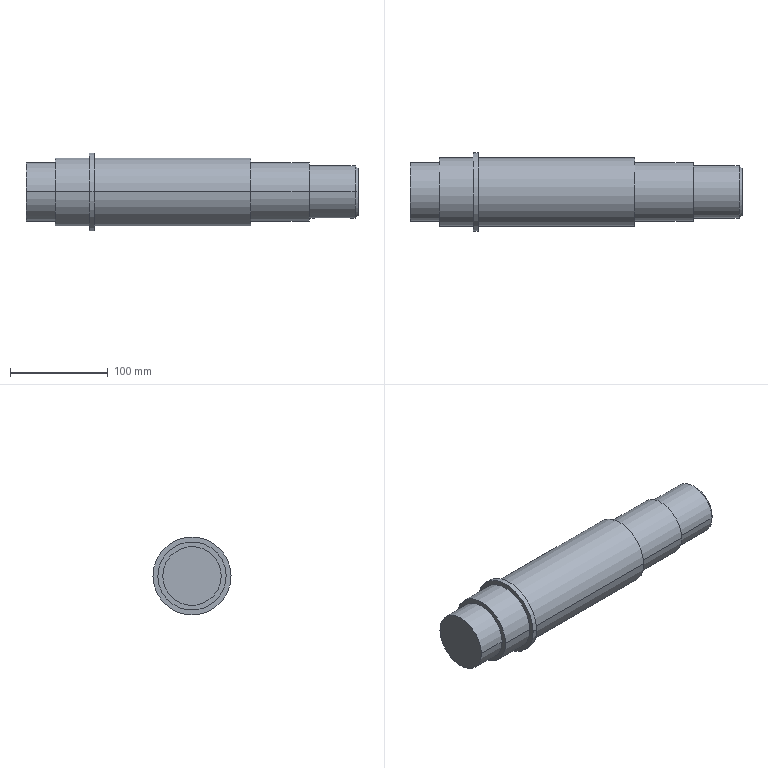Component | SolidWorks | TurbineShaft-1 | 1 solid | 28 faces | box 340 x 80 x 80 mm | volume 1142290 mm3 | cylinder 16 | plane 10 | cone 2 | commonest cylinder face diameters 60 x4 70 x4 10 x4 54 x2 80 x2
STEP:
#1=COLOUR_RGB('',0.7922,0.8196,0.9333);
#2=FILL_AREA_STYLE_COLOUR('',#1);
#3=FILL_AREA_STYLE('',(#2));
#4=SURFACE_STYLE_FILL_AREA(#3);
#5=SURFACE_SIDE_STYLE('',(#4));
#6=SURFACE_STYLE_USAGE(.BOTH.,#5);
#7=PRESENTATION_STYLE_ASSIGNMENT((#6));
#8=CARTESIAN_POINT('',(6.676,-1.282,-6.483));
#9=VERTEX_POINT('',#8);
#10=CARTESIAN_POINT('',(6.676,0.6077,-6.509));
#11=VERTEX_POINT('',#10);
#12=CARTESIAN_POINT('',(6.676,-0.3371,-6.496));
#13=DIRECTION('',(1.,0.,0.));
#14=DIRECTION('',(0.,0.9999,-0.01398));
#15=AXIS2_PLACEMENT_3D('',#12,#13,#14);
#16=CIRCLE('',#15,0.9449);
#17=EDGE_CURVE('',#9,#11,#16,.T.);
#18=ORIENTED_EDGE('',*,*,#17,.F.);
#19=CARTESIAN_POINT('',(6.558,-1.4,-6.481));
#20=VERTEX_POINT('',#19);
#21=CARTESIAN_POINT('',(6.558,-1.4,-6.481));
#22=DIRECTION('',(-0.7071,-0.707,0.009885));
#23=VECTOR('',#22,39.37);
#24=LINE('',#21,#23);
#25=EDGE_CURVE('',#9,#20,#24,.T.);
#26=ORIENTED_EDGE('',*,*,#25,.T.);
#27=CARTESIAN_POINT('',(6.558,0.7258,-6.511));
#28=VERTEX_POINT('',#27);
#29=CARTESIAN_POINT('',(6.558,-0.3371,-6.496));
#30=DIRECTION('',(-1.,-0.,-0.));
#31=DIRECTION('',(0.,0.9999,-0.01398));
#32=AXIS2_PLACEMENT_3D('',#29,#30,#31);
#33=CIRCLE('',#32,1.063);
#34=EDGE_CURVE('',#28,#20,#33,.T.);
#35=ORIENTED_EDGE('',*,*,#34,.F.);
#36=CARTESIAN_POINT('',(6.558,0.7258,-6.511));
#37=DIRECTION('',(-0.7071,0.707,-0.009885));
#38=VECTOR('',#37,39.37);
#39=LINE('',#36,#38);
#40=EDGE_CURVE('',#11,#28,#39,.T.);
#41=ORIENTED_EDGE('',*,*,#40,.F.);
#42=EDGE_LOOP('',(#18,#26,#35,#41));
#43=FACE_OUTER_BOUND('',#42,.T.);
#44=CARTESIAN_POINT('',(6.558,-0.3371,-6.496));
#45=DIRECTION('',(-1.,-0.,-0.));
#46=DIRECTION('',(0.,0.9999,-0.01398));
#47=AXIS2_PLACEMENT_3D('',#44,#45,#46);
#48=CONICAL_SURFACE('',#47,1.063,0.7854);
#49=ADVANCED_FACE('',(#43),#48,.T.);
#50=CARTESIAN_POINT('',(6.282,-0.5485,-7.538));
#51=VERTEX_POINT('',#50);
#52=CARTESIAN_POINT('',(6.479,-0.3519,-7.559));
#53=VERTEX_POINT('',#52);
#54=CARTESIAN_POINT('',(6.282,-0.5485,-7.538));
#55=CARTESIAN_POINT('',(6.295,-0.5485,-7.538));
#56=CARTESIAN_POINT('',(6.308,-0.5472,-7.538));
#57=CARTESIAN_POINT('',(6.327,-0.5435,-7.539));
#58=CARTESIAN_POINT('',(6.333,-0.5419,-7.539));
#59=CARTESIAN_POINT('',(6.346,-0.5382,-7.54));
#60=CARTESIAN_POINT('',(6.352,-0.536,-7.54));
#61=CARTESIAN_POINT('',(6.37,-0.5286,-7.542));
#62=CARTESIAN_POINT('',(6.381,-0.5226,-7.543));
#63=CARTESIAN_POINT('',(6.402,-0.5083,-7.545));
#64=CARTESIAN_POINT('',(6.412,-0.5001,-7.547));
#65=CARTESIAN_POINT('',(6.431,-0.482,-7.549));
#66=CARTESIAN_POINT('',(6.439,-0.4721,-7.55));
#67=CARTESIAN_POINT('',(6.453,-0.4507,-7.553));
#68=CARTESIAN_POINT('',(6.459,-0.4393,-7.554));
#69=CARTESIAN_POINT('',(6.469,-0.4157,-7.556));
#70=CARTESIAN_POINT('',(6.473,-0.4033,-7.557));
#71=CARTESIAN_POINT('',(6.478,-0.3778,-7.558));
#72=CARTESIAN_POINT('',(6.479,-0.3649,-7.559));
#73=CARTESIAN_POINT('',(6.479,-0.3519,-7.559));
#74=B_SPLINE_CURVE_WITH_KNOTS('',3,(#54,#55,#56,#57,#58,#59,#60,#61,#62,#63,#64,#65,#66,#67,#68,#69,#70,#71,#72,#73),.UNSPECIFIED.,.F.,.F.,(4,2,2,2,2,2,2,2,2,4),(0.,0.0009785,0.001468,0.001957,0.002935,0.003914,0.004892,0.005871,0.006849,0.007828),.UNSPECIFIED.);
#75=EDGE_CURVE('',#51,#53,#74,.T.);
#76=ORIENTED_EDGE('',*,*,#75,.T.);
#77=CARTESIAN_POINT('',(6.282,-0.1548,-7.543));
#78=VERTEX_POINT('',#77);
#79=CARTESIAN_POINT('',(6.479,-0.3519,-7.559));
#80=CARTESIAN_POINT('',(6.479,-0.3389,-7.559));
#81=CARTESIAN_POINT('',(6.478,-0.3261,-7.559));
#82=CARTESIAN_POINT('',(6.474,-0.3072,-7.559));
#83=CARTESIAN_POINT('',(6.473,-0.3009,-7.558));
#84=CARTESIAN_POINT('',(6.469,-0.2886,-7.558));
#85=CARTESIAN_POINT('',(6.467,-0.2824,-7.558));
#86=CARTESIAN_POINT('',(6.459,-0.2645,-7.557));
#87=CARTESIAN_POINT('',(6.453,-0.2532,-7.556));
#88=CARTESIAN_POINT('',(6.439,-0.2318,-7.554));
#89=CARTESIAN_POINT('',(6.431,-0.2217,-7.553));
#90=CARTESIAN_POINT('',(6.413,-0.2036,-7.551));
#91=CARTESIAN_POINT('',(6.403,-0.1954,-7.55));
#92=CARTESIAN_POINT('',(6.381,-0.181,-7.548));
#93=CARTESIAN_POINT('',(6.37,-0.1749,-7.547));
#94=CARTESIAN_POINT('',(6.346,-0.165,-7.545));
#95=CARTESIAN_POINT('',(6.334,-0.1612,-7.544));
#96=CARTESIAN_POINT('',(6.308,-0.1561,-7.544));
#97=CARTESIAN_POINT('',(6.295,-0.1548,-7.543));
#98=CARTESIAN_POINT('',(6.282,-0.1548,-7.543));
#99=B_SPLINE_CURVE_WITH_KNOTS('',3,(#79,#80,#81,#82,#83,#84,#85,#86,#87,#88,#89,#90,#91,#92,#93,#94,#95,#96,#97,#98),.UNSPECIFIED.,.F.,.F.,(4,2,2,2,2,2,2,2,2,4),(0.,0.0009785,0.001468,0.001957,0.002935,0.003914,0.004892,0.005871,0.006849,0.007828),.UNSPECIFIED.);
#100=EDGE_CURVE('',#53,#78,#99,.T.);
#101=ORIENTED_EDGE('',*,*,#100,.T.);
#102=CARTESIAN_POINT('',(5.022,-0.1548,-7.543));
#103=VERTEX_POINT('',#102);
#104=CARTESIAN_POINT('',(-6.71,-0.1548,-7.543));
#105=DIRECTION('',(-1.,-0.,-0.));
#106=VECTOR('',#105,39.37);
#107=LINE('',#104,#106);
#108=EDGE_CURVE('',#78,#103,#107,.T.);
#109=ORIENTED_EDGE('',*,*,#108,.T.);
#110=CARTESIAN_POINT('',(4.826,-0.3519,-7.559));
#111=VERTEX_POINT('',#110);
#112=CARTESIAN_POINT('',(5.022,-0.1548,-7.543));
#113=CARTESIAN_POINT('',(5.009,-0.1548,-7.543));
#114=CARTESIAN_POINT('',(4.997,-0.1561,-7.544));
#115=CARTESIAN_POINT('',(4.978,-0.1599,-7.544));
#116=CARTESIAN_POINT('',(4.972,-0.1615,-7.544));
#117=CARTESIAN_POINT('',(4.959,-0.1652,-7.545));
#118=CARTESIAN_POINT('',(4.953,-0.1674,-7.545));
#119=CARTESIAN_POINT('',(4.935,-0.1748,-7.547));
#120=CARTESIAN_POINT('',(4.924,-0.1809,-7.548));
#121=CARTESIAN_POINT('',(4.902,-0.1952,-7.55));
#122=CARTESIAN_POINT('',(4.892,-0.2035,-7.551));
#123=CARTESIAN_POINT('',(4.874,-0.2216,-7.553));
#124=CARTESIAN_POINT('',(4.866,-0.2315,-7.554));
#125=CARTESIAN_POINT('',(4.852,-0.253,-7.556));
#126=CARTESIAN_POINT('',(4.846,-0.2645,-7.557));
#127=CARTESIAN_POINT('',(4.836,-0.2881,-7.558));
#128=CARTESIAN_POINT('',(4.832,-0.3006,-7.559));
#129=CARTESIAN_POINT('',(4.827,-0.326,-7.559));
#130=CARTESIAN_POINT('',(4.826,-0.3389,-7.559));
#131=CARTESIAN_POINT('',(4.826,-0.3519,-7.559));
#132=B_SPLINE_CURVE_WITH_KNOTS('',3,(#112,#113,#114,#115,#116,#117,#118,#119,#120,#121,#122,#123,#124,#125,#126,#127,#128,#129,#130,#131),.UNSPECIFIED.,.F.,.F.,(4,2,2,2,2,2,2,2,2,4),(0.,0.0009785,0.001468,0.001957,0.002935,0.003914,0.004892,0.005871,0.006849,0.007828),.UNSPECIFIED.);
#133=EDGE_CURVE('',#103,#111,#132,.T.);
#134=ORIENTED_EDGE('',*,*,#133,.T.);
#135=CARTESIAN_POINT('',(5.022,-0.5485,-7.538));
#136=VERTEX_POINT('',#135);
#137=CARTESIAN_POINT('',(4.826,-0.3519,-7.559));
#138=CARTESIAN_POINT('',(4.826,-0.3649,-7.559));
#139=CARTESIAN_POINT('',(4.827,-0.3777,-7.558));
#140=CARTESIAN_POINT('',(4.831,-0.3966,-7.557));
#141=CARTESIAN_POINT('',(4.832,-0.4029,-7.557));
#142=CARTESIAN_POINT('',(4.836,-0.4152,-7.556));
#143=CARTESIAN_POINT('',(4.838,-0.4214,-7.556));
#144=CARTESIAN_POINT('',(4.846,-0.4392,-7.554));
#145=CARTESIAN_POINT('',(4.852,-0.4505,-7.553));
#146=CARTESIAN_POINT('',(4.866,-0.4718,-7.551));
#147=CARTESIAN_POINT('',(4.874,-0.4819,-7.549));
#148=CARTESIAN_POINT('',(4.892,-0.5,-7.547));
#149=CARTESIAN_POINT('',(4.902,-0.5081,-7.545));
#150=CARTESIAN_POINT('',(4.924,-0.5225,-7.543));
#151=CARTESIAN_POINT('',(4.935,-0.5285,-7.542));
#152=CARTESIAN_POINT('',(4.959,-0.5384,-7.54));
#153=CARTESIAN_POINT('',(4.971,-0.5421,-7.539));
#154=CARTESIAN_POINT('',(4.997,-0.5472,-7.538));
#155=CARTESIAN_POINT('',(5.009,-0.5485,-7.538));
#156=CARTESIAN_POINT('',(5.022,-0.5485,-7.538));
#157=B_SPLINE_CURVE_WITH_KNOTS('',3,(#137,#138,#139,#140,#141,#142,#143,#144,#145,#146,#147,#148,#149,#150,#151,#152,#153,#154,#155,#156),.UNSPECIFIED.,.F.,.F.,(4,2,2,2,2,2,2,2,2,4),(0.,0.0009785,0.001468,0.001957,0.002935,0.003914,0.004892,0.005871,0.006849,0.007828),.UNSPECIFIED.);
#158=EDGE_CURVE('',#111,#136,#157,.T.);
#159=ORIENTED_EDGE('',*,*,#158,.T.);
#160=CARTESIAN_POINT('',(-6.71,-0.5485,-7.538));
#161=DIRECTION('',(1.,0.,0.));
#162=VECTOR('',#161,39.37);
#163=LINE('',#160,#162);
#164=EDGE_CURVE('',#136,#51,#163,.T.);
#165=ORIENTED_EDGE('',*,*,#164,.T.);
#166=EDGE_LOOP('',(#76,#101,#109,#134,#159,#165));
#167=FACE_BOUND('',#166,.T.);
#168=ORIENTED_EDGE('',*,*,#34,.T.);
#169=CARTESIAN_POINT('',(4.708,-1.4,-6.481));
#170=VERTEX_POINT('',#169);
#171=CARTESIAN_POINT('',(-6.71,-1.4,-6.481));
#172=DIRECTION('',(-1.,-0.,-0.));
#173=VECTOR('',#172,39.37);
#174=LINE('',#171,#173);
#175=EDGE_CURVE('',#20,#170,#174,.T.);
#176=ORIENTED_EDGE('',*,*,#175,.T.);
#177=CARTESIAN_POINT('',(4.708,0.7258,-6.511));
#178=VERTEX_POINT('',#177);
#179=CARTESIAN_POINT('',(4.708,-0.3371,-6.496));
#180=DIRECTION('',(-1.,-0.,-0.));
#181=DIRECTION('',(0.,0.9999,-0.01398));
#182=AXIS2_PLACEMENT_3D('',#179,#180,#181);
#183=CIRCLE('',#182,1.063);
#184=EDGE_CURVE('',#178,#170,#183,.T.);
#185=ORIENTED_EDGE('',*,*,#184,.F.);
#186=CARTESIAN_POINT('',(-6.71,0.7258,-6.511));
#187=DIRECTION('',(-1.,-0.,-0.));
#188=VECTOR('',#187,39.37);
#189=LINE('',#186,#188);
#190=EDGE_CURVE('',#28,#178,#189,.T.);
#191=ORIENTED_EDGE('',*,*,#190,.F.);
#192=EDGE_LOOP('',(#168,#176,#185,#191));
#193=FACE_OUTER_BOUND('',#192,.T.);
#194=CARTESIAN_POINT('',(-6.71,-0.3371,-6.496));
#195=DIRECTION('',(-1.,-0.,-0.));
#196=DIRECTION('',(0.,0.9999,-0.01398));
#197=AXIS2_PLACEMENT_3D('',#194,#195,#196);
#198=CYLINDRICAL_SURFACE('',#197,1.063);
#199=ADVANCED_FACE('',(#167,#193),#198,.T.);
#200=CARTESIAN_POINT('',(4.708,0.8439,-6.513));
#201=VERTEX_POINT('',#200);
#202=CARTESIAN_POINT('',(4.708,-1.518,-6.48));
#203=VERTEX_POINT('',#202);
#204=CARTESIAN_POINT('',(4.708,-0.3371,-6.496));
#205=DIRECTION('',(-1.,-0.,-0.));
#206=DIRECTION('',(0.,0.9999,-0.01398));
#207=AXIS2_PLACEMENT_3D('',#204,#205,#206);
#208=CIRCLE('',#207,1.181);
#209=EDGE_CURVE('',#201,#203,#208,.T.);
#210=ORIENTED_EDGE('',*,*,#209,.T.);
#211=CARTESIAN_POINT('',(2.345,-1.518,-6.48));
#212=VERTEX_POINT('',#211);
#213=CARTESIAN_POINT('',(-6.71,-1.518,-6.48));
#214=DIRECTION('',(-1.,-0.,-0.));
#215=VECTOR('',#214,39.37);
#216=LINE('',#213,#215);
#217=EDGE_CURVE('',#203,#212,#216,.T.);
#218=ORIENTED_EDGE('',*,*,#217,.T.);
#219=CARTESIAN_POINT('',(2.345,0.8439,-6.513));
#220=VERTEX_POINT('',#219);
#221=CARTESIAN_POINT('',(2.345,-0.3371,-6.496));
#222=DIRECTION('',(-1.,-0.,-0.));
#223=DIRECTION('',(0.,0.9999,-0.01398));
#224=AXIS2_PLACEMENT_3D('',#221,#222,#223);
#225=CIRCLE('',#224,1.181);
#226=EDGE_CURVE('',#220,#212,#225,.T.);
#227=ORIENTED_EDGE('',*,*,#226,.F.);
#228=CARTESIAN_POINT('',(-6.71,0.8439,-6.513));
#229=DIRECTION('',(-1.,-0.,-0.));
#230=VECTOR('',#229,39.37);
#231=LINE('',#228,#230);
#232=EDGE_CURVE('',#201,#220,#231,.T.);
#233=ORIENTED_EDGE('',*,*,#232,.F.);
#234=EDGE_LOOP('',(#210,#218,#227,#233));
#235=FACE_OUTER_BOUND('',#234,.T.);
#236=CARTESIAN_POINT('',(-6.71,-0.3371,-6.496));
#237=DIRECTION('',(-1.,-0.,-0.));
#238=DIRECTION('',(0.,0.9999,-0.01398));
#239=AXIS2_PLACEMENT_3D('',#236,#237,#238);
#240=CYLINDRICAL_SURFACE('',#239,1.181);
#241=ADVANCED_FACE('',(#235),#240,.T.);
#242=CARTESIAN_POINT('',(2.345,1.041,-6.515));
#243=VERTEX_POINT('',#242);
#244=CARTESIAN_POINT('',(2.345,-1.715,-6.477));
#245=VERTEX_POINT('',#244);
#246=CARTESIAN_POINT('',(2.345,-0.3371,-6.496));
#247=DIRECTION('',(-1.,-0.,-0.));
#248=DIRECTION('',(-0.,0.9999,-0.01398));
#249=AXIS2_PLACEMENT_3D('',#246,#247,#248);
#250=CIRCLE('',#249,1.378);
#251=EDGE_CURVE('',#243,#245,#250,.T.);
#252=ORIENTED_EDGE('',*,*,#251,.T.);
#253=CARTESIAN_POINT('',(-3.954,-1.715,-6.477));
#254=VERTEX_POINT('',#253);
#255=CARTESIAN_POINT('',(-6.71,-1.715,-6.477));
#256=DIRECTION('',(-1.,-0.,-0.));
#257=VECTOR('',#256,39.37);
#258=LINE('',#255,#257);
#259=EDGE_CURVE('',#245,#254,#258,.T.);
#260=ORIENTED_EDGE('',*,*,#259,.T.);
#261=CARTESIAN_POINT('',(-3.954,1.041,-6.515));
#262=VERTEX_POINT('',#261);
#263=CARTESIAN_POINT('',(-3.954,-0.3371,-6.496));
#264=DIRECTION('',(-1.,-0.,-0.));
#265=DIRECTION('',(0.,0.9999,-0.01398));
#266=AXIS2_PLACEMENT_3D('',#263,#264,#265);
#267=CIRCLE('',#266,1.378);
#268=EDGE_CURVE('',#262,#254,#267,.T.);
#269=ORIENTED_EDGE('',*,*,#268,.F.);
#270=CARTESIAN_POINT('',(-6.71,1.041,-6.515));
#271=DIRECTION('',(-1.,-0.,-0.));
#272=VECTOR('',#271,39.37);
#273=LINE('',#270,#272);
#274=EDGE_CURVE('',#243,#262,#273,.T.);
#275=ORIENTED_EDGE('',*,*,#274,.F.);
#276=EDGE_LOOP('',(#252,#260,#269,#275));
#277=FACE_OUTER_BOUND('',#276,.T.);
#278=CARTESIAN_POINT('',(-6.71,-0.3371,-6.496));
#279=DIRECTION('',(-1.,-0.,-0.));
#280=DIRECTION('',(0.,0.9999,-0.01398));
#281=AXIS2_PLACEMENT_3D('',#278,#279,#280);
#282=CYLINDRICAL_SURFACE('',#281,1.378);
#283=ADVANCED_FACE('',(#277),#282,.T.);
#284=CARTESIAN_POINT('',(-3.954,1.238,-6.518));
#285=VERTEX_POINT('',#284);
#286=CARTESIAN_POINT('',(-3.954,-1.912,-6.474));
#287=VERTEX_POINT('',#286);
#288=CARTESIAN_POINT('',(-3.954,-0.3371,-6.496));
#289=DIRECTION('',(-1.,-0.,-0.));
#290=DIRECTION('',(0.,0.9999,-0.01398));
#291=AXIS2_PLACEMENT_3D('',#288,#289,#290);
#292=CIRCLE('',#291,1.575);
#293=EDGE_CURVE('',#285,#287,#292,.T.);
#294=ORIENTED_EDGE('',*,*,#293,.T.);
#295=CARTESIAN_POINT('',(-4.151,-1.912,-6.474));
#296=VERTEX_POINT('',#295);
#297=CARTESIAN_POINT('',(-6.71,-1.912,-6.474));
#298=DIRECTION('',(-1.,-0.,-0.));
#299=VECTOR('',#298,39.37);
#300=LINE('',#297,#299);
#301=EDGE_CURVE('',#287,#296,#300,.T.);
#302=ORIENTED_EDGE('',*,*,#301,.T.);
#303=CARTESIAN_POINT('',(-4.151,1.238,-6.518));
#304=VERTEX_POINT('',#303);
#305=CARTESIAN_POINT('',(-4.151,-0.3371,-6.496));
#306=DIRECTION('',(-1.,-0.,-0.));
#307=DIRECTION('',(0.,0.9999,-0.01398));
#308=AXIS2_PLACEMENT_3D('',#305,#306,#307);
#309=CIRCLE('',#308,1.575);
#310=EDGE_CURVE('',#304,#296,#309,.T.);
#311=ORIENTED_EDGE('',*,*,#310,.F.);
#312=CARTESIAN_POINT('',(-6.71,1.238,-6.518));
#313=DIRECTION('',(-1.,-0.,-0.));
#314=VECTOR('',#313,39.37);
#315=LINE('',#312,#314);
#316=EDGE_CURVE('',#285,#304,#315,.T.);
#317=ORIENTED_EDGE('',*,*,#316,.F.);
#318=EDGE_LOOP('',(#294,#302,#311,#317));
#319=FACE_OUTER_BOUND('',#318,.T.);
#320=CARTESIAN_POINT('',(-6.71,-0.3371,-6.496));
#321=DIRECTION('',(-1.,-0.,-0.));
#322=DIRECTION('',(0.,0.9999,-0.01398));
#323=AXIS2_PLACEMENT_3D('',#320,#321,#322);
#324=CYLINDRICAL_SURFACE('',#323,1.575);
#325=ADVANCED_FACE('',(#319),#324,.T.);
#326=CARTESIAN_POINT('',(-4.151,1.041,-6.515));
#327=VERTEX_POINT('',#326);
#328=CARTESIAN_POINT('',(-4.151,-1.715,-6.477));
#329=VERTEX_POINT('',#328);
#330=CARTESIAN_POINT('',(-4.151,-0.3371,-6.496));
#331=DIRECTION('',(-1.,-0.,-0.));
#332=DIRECTION('',(0.,0.9999,-0.01398));
#333=AXIS2_PLACEMENT_3D('',#330,#331,#332);
#334=CIRCLE('',#333,1.378);
#335=EDGE_CURVE('',#327,#329,#334,.T.);
#336=ORIENTED_EDGE('',*,*,#335,.T.);
#337=CARTESIAN_POINT('',(-5.529,-1.715,-6.477));
#338=VERTEX_POINT('',#337);
#339=CARTESIAN_POINT('',(-6.71,-1.715,-6.477));
#340=DIRECTION('',(-1.,-0.,-0.));
#341=VECTOR('',#340,39.37);
#342=LINE('',#339,#341);
#343=EDGE_CURVE('',#329,#338,#342,.T.);
#344=ORIENTED_EDGE('',*,*,#343,.T.);
#345=CARTESIAN_POINT('',(-5.529,1.041,-6.515));
#346=VERTEX_POINT('',#345);
#347=CARTESIAN_POINT('',(-5.529,-0.3371,-6.496));
#348=DIRECTION('',(-1.,-0.,-0.));
#349=DIRECTION('',(0.,0.9999,-0.01398));
#350=AXIS2_PLACEMENT_3D('',#347,#348,#349);
#351=CIRCLE('',#350,1.378);
#352=EDGE_CURVE('',#346,#338,#351,.T.);
#353=ORIENTED_EDGE('',*,*,#352,.F.);
#354=CARTESIAN_POINT('',(-6.71,1.041,-6.515));
#355=DIRECTION('',(-1.,-0.,-0.));
#356=VECTOR('',#355,39.37);
#357=LINE('',#354,#356);
#358=EDGE_CURVE('',#327,#346,#357,.T.);
#359=ORIENTED_EDGE('',*,*,#358,.F.);
#360=EDGE_LOOP('',(#336,#344,#353,#359));
#361=FACE_OUTER_BOUND('',#360,.T.);
#362=CARTESIAN_POINT('',(-6.71,-0.3371,-6.496));
#363=DIRECTION('',(-1.,-0.,-0.));
#364=DIRECTION('',(0.,0.9999,-0.01398));
#365=AXIS2_PLACEMENT_3D('',#362,#363,#364);
#366=CYLINDRICAL_SURFACE('',#365,1.378);
#367=ADVANCED_FACE('',(#361),#366,.T.);
#368=CARTESIAN_POINT('',(-5.529,0.8439,-6.513));
#369=VERTEX_POINT('',#368);
#370=CARTESIAN_POINT('',(-5.529,-1.518,-6.48));
#371=VERTEX_POINT('',#370);
#372=CARTESIAN_POINT('',(-5.529,-0.3371,-6.496));
#373=DIRECTION('',(-1.,-0.,-0.));
#374=DIRECTION('',(0.,0.9999,-0.01398));
#375=AXIS2_PLACEMENT_3D('',#372,#373,#374);
#376=CIRCLE('',#375,1.181);
#377=EDGE_CURVE('',#369,#371,#376,.T.);
#378=ORIENTED_EDGE('',*,*,#377,.T.);
#379=CARTESIAN_POINT('',(-6.71,-1.518,-6.48));
#380=VERTEX_POINT('',#379);
#381=CARTESIAN_POINT('',(-6.71,-1.518,-6.48));
#382=DIRECTION('',(-1.,-0.,-0.));
#383=VECTOR('',#382,39.37);
#384=LINE('',#381,#383);
#385=EDGE_CURVE('',#371,#380,#384,.T.);
#386=ORIENTED_EDGE('',*,*,#385,.T.);
#387=CARTESIAN_POINT('',(-6.71,0.8439,-6.513));
#388=VERTEX_POINT('',#387);
#389=CARTESIAN_POINT('',(-6.71,-0.3371,-6.496));
#390=DIRECTION('',(-1.,-0.,-0.));
#391=DIRECTION('',(0.,0.9999,-0.01398));
#392=AXIS2_PLACEMENT_3D('',#389,#390,#391);
#393=CIRCLE('',#392,1.181);
#394=EDGE_CURVE('',#388,#380,#393,.T.);
#395=ORIENTED_EDGE('',*,*,#394,.F.);
#396=CARTESIAN_POINT('',(-6.71,0.8439,-6.513));
#397=DIRECTION('',(-1.,-0.,-0.));
#398=VECTOR('',#397,39.37);
#399=LINE('',#396,#398);
#400=EDGE_CURVE('',#369,#388,#399,.T.);
#401=ORIENTED_EDGE('',*,*,#400,.F.);
#402=EDGE_LOOP('',(#378,#386,#395,#401));
#403=FACE_OUTER_BOUND('',#402,.T.);
#404=CARTESIAN_POINT('',(-6.71,-0.3371,-6.496));
#405=DIRECTION('',(-1.,-0.,-0.));
#406=DIRECTION('',(0.,0.9999,-0.01398));
#407=AXIS2_PLACEMENT_3D('',#404,#405,#406);
#408=CYLINDRICAL_SURFACE('',#407,1.181);
#409=ADVANCED_FACE('',(#403),#408,.T.);
#410=ORIENTED_EDGE('',*,*,#394,.T.);
#411=CARTESIAN_POINT('',(-6.71,-0.3371,-6.496));
#412=DIRECTION('',(-1.,-0.,-0.));
#413=DIRECTION('',(0.,0.9999,-0.01398));
#414=AXIS2_PLACEMENT_3D('',#411,#412,#413);
#415=CIRCLE('',#414,1.181);
#416=EDGE_CURVE('',#380,#388,#415,.T.);
#417=ORIENTED_EDGE('',*,*,#416,.T.);
#418=EDGE_LOOP('',(#410,#417));
#419=FACE_OUTER_BOUND('',#418,.T.);
#420=CARTESIAN_POINT('',(-6.71,-0.3371,-6.496));
#421=DIRECTION('',(1.,0.,0.));
#422=DIRECTION('',(0.,-0.9999,0.01398));
#423=AXIS2_PLACEMENT_3D('',#420,#421,#422);
#424=PLANE('',#423);
#425=ADVANCED_FACE('',(#419),#424,.F.);
#426=ORIENTED_EDGE('',*,*,#385,.F.);
#427=CARTESIAN_POINT('',(-5.529,-0.3371,-6.496));
#428=DIRECTION('',(-1.,-0.,-0.));
#429=DIRECTION('',(0.,0.9999,-0.01398));
#430=AXIS2_PLACEMENT_3D('',#427,#428,#429);
#431=CIRCLE('',#430,1.181);
#432=EDGE_CURVE('',#371,#369,#431,.T.);
#433=ORIENTED_EDGE('',*,*,#432,.T.);
#434=ORIENTED_EDGE('',*,*,#400,.T.);
#435=ORIENTED_EDGE('',*,*,#416,.F.);
#436=EDGE_LOOP('',(#426,#433,#434,#435));
#437=FACE_OUTER_BOUND('',#436,.T.);
#438=CARTESIAN_POINT('',(-6.71,-0.3371,-6.496));
#439=DIRECTION('',(-1.,-0.,-0.));
#440=DIRECTION('',(0.,0.9999,-0.01398));
#441=AXIS2_PLACEMENT_3D('',#438,#439,#440);
#442=CYLINDRICAL_SURFACE('',#441,1.181);
#443=ADVANCED_FACE('',(#437),#442,.T.);
#444=ORIENTED_EDGE('',*,*,#377,.F.);
#445=ORIENTED_EDGE('',*,*,#432,.F.);
#446=EDGE_LOOP('',(#444,#445));
#447=FACE_BOUND('',#446,.T.);
#448=ORIENTED_EDGE('',*,*,#352,.T.);
#449=CARTESIAN_POINT('',(-5.529,-0.3371,-6.496));
#450=DIRECTION('',(-1.,-0.,-0.));
#451=DIRECTION('',(0.,0.9999,-0.01398));
#452=AXIS2_PLACEMENT_3D('',#449,#450,#451);
#453=CIRCLE('',#452,1.378);
#454=EDGE_CURVE('',#338,#346,#453,.T.);
#455=ORIENTED_EDGE('',*,*,#454,.T.);
#456=EDGE_LOOP('',(#448,#455));
#457=FACE_OUTER_BOUND('',#456,.T.);
#458=CARTESIAN_POINT('',(-5.529,-1.518,-6.48));
#459=DIRECTION('',(1.,0.,0.));
#460=DIRECTION('',(0.,-0.9999,0.01398));
#461=AXIS2_PLACEMENT_3D('',#458,#459,#460);
#462=PLANE('',#461);
#463=ADVANCED_FACE('',(#447,#457),#462,.F.);
#464=ORIENTED_EDGE('',*,*,#343,.F.);
#465=CARTESIAN_POINT('',(-4.151,-0.3371,-6.496));
#466=DIRECTION('',(-1.,-0.,-0.));
#467=DIRECTION('',(0.,0.9999,-0.01398));
#468=AXIS2_PLACEMENT_3D('',#465,#466,#467);
#469=CIRCLE('',#468,1.378);
#470=EDGE_CURVE('',#329,#327,#469,.T.);
#471=ORIENTED_EDGE('',*,*,#470,.T.);
#472=ORIENTED_EDGE('',*,*,#358,.T.);
#473=ORIENTED_EDGE('',*,*,#454,.F.);
#474=EDGE_LOOP('',(#464,#471,#472,#473));
#475=FACE_OUTER_BOUND('',#474,.T.);
#476=CARTESIAN_POINT('',(-6.71,-0.3371,-6.496));
#477=DIRECTION('',(-1.,-0.,-0.));
#478=DIRECTION('',(0.,0.9999,-0.01398));
#479=AXIS2_PLACEMENT_3D('',#476,#477,#478);
#480=CYLINDRICAL_SURFACE('',#479,1.378);
#481=ADVANCED_FACE('',(#475),#480,.T.);
#482=ORIENTED_EDGE('',*,*,#335,.F.);
#483=ORIENTED_EDGE('',*,*,#470,.F.);
#484=EDGE_LOOP('',(#482,#483));
#485=FACE_BOUND('',#484,.T.);
#486=ORIENTED_EDGE('',*,*,#310,.T.);
#487=CARTESIAN_POINT('',(-4.151,-0.3371,-6.496));
#488=DIRECTION('',(-1.,-0.,-0.));
#489=DIRECTION('',(0.,0.9999,-0.01398));
#490=AXIS2_PLACEMENT_3D('',#487,#488,#489);
#491=CIRCLE('',#490,1.575);
#492=EDGE_CURVE('',#296,#304,#491,.T.);
#493=ORIENTED_EDGE('',*,*,#492,.T.);
#494=EDGE_LOOP('',(#486,#493));
#495=FACE_OUTER_BOUND('',#494,.T.);
#496=CARTESIAN_POINT('',(-4.151,-1.715,-6.477));
#497=DIRECTION('',(1.,0.,0.));
#498=DIRECTION('',(0.,-0.9999,0.01398));
#499=AXIS2_PLACEMENT_3D('',#496,#497,#498);
#500=PLANE('',#499);
#501=ADVANCED_FACE('',(#485,#495),#500,.F.);
#502=ORIENTED_EDGE('',*,*,#301,.F.);
#503=CARTESIAN_POINT('',(-3.954,-0.3371,-6.496));
#504=DIRECTION('',(-1.,-0.,-0.));
#505=DIRECTION('',(0.,0.9999,-0.01398));
#506=AXIS2_PLACEMENT_3D('',#503,#504,#505);
#507=CIRCLE('',#506,1.575);
#508=EDGE_CURVE('',#287,#285,#507,.T.);
#509=ORIENTED_EDGE('',*,*,#508,.T.);
#510=ORIENTED_EDGE('',*,*,#316,.T.);
#511=ORIENTED_EDGE('',*,*,#492,.F.);
#512=EDGE_LOOP('',(#502,#509,#510,#511));
#513=FACE_OUTER_BOUND('',#512,.T.);
#514=CARTESIAN_POINT('',(-6.71,-0.3371,-6.496));
#515=DIRECTION('',(-1.,-0.,-0.));
#516=DIRECTION('',(0.,0.9999,-0.01398));
#517=AXIS2_PLACEMENT_3D('',#514,#515,#516);
#518=CYLINDRICAL_SURFACE('',#517,1.575);
#519=ADVANCED_FACE('',(#513),#518,.T.);
#520=ORIENTED_EDGE('',*,*,#293,.F.);
#521=ORIENTED_EDGE('',*,*,#508,.F.);
#522=EDGE_LOOP('',(#520,#521));
#523=FACE_OUTER_BOUND('',#522,.T.);
#524=ORIENTED_EDGE('',*,*,#268,.T.);
#525=CARTESIAN_POINT('',(-3.954,-0.3371,-6.496));
#526=DIRECTION('',(-1.,-0.,-0.));
#527=DIRECTION('',(0.,0.9999,-0.01398));
#528=AXIS2_PLACEMENT_3D('',#525,#526,#527);
#529=CIRCLE('',#528,1.378);
#530=EDGE_CURVE('',#254,#262,#529,.T.);
#531=ORIENTED_EDGE('',*,*,#530,.T.);
#532=EDGE_LOOP('',(#524,#531));
#533=FACE_BOUND('',#532,.T.);
#534=CARTESIAN_POINT('',(-3.954,-1.912,-6.474));
#535=DIRECTION('',(-1.,-0.,-0.));
#536=DIRECTION('',(-0.,0.9999,-0.01398));
#537=AXIS2_PLACEMENT_3D('',#534,#535,#536);
#538=PLANE('',#537);
#539=ADVANCED_FACE('',(#523,#533),#538,.F.);
#540=ORIENTED_EDGE('',*,*,#259,.F.);
#541=CARTESIAN_POINT('',(2.345,-0.3371,-6.496));
#542=DIRECTION('',(-1.,-0.,-0.));
#543=DIRECTION('',(-0.,0.9999,-0.01398));
#544=AXIS2_PLACEMENT_3D('',#541,#542,#543);
#545=CIRCLE('',#544,1.378);
#546=EDGE_CURVE('',#245,#243,#545,.T.);
#547=ORIENTED_EDGE('',*,*,#546,.T.);
#548=ORIENTED_EDGE('',*,*,#274,.T.);
#549=ORIENTED_EDGE('',*,*,#530,.F.);
#550=EDGE_LOOP('',(#540,#547,#548,#549));
#551=FACE_OUTER_BOUND('',#550,.T.);
#552=CARTESIAN_POINT('',(-6.71,-0.3371,-6.496));
#553=DIRECTION('',(-1.,-0.,-0.));
#554=DIRECTION('',(0.,0.9999,-0.01398));
#555=AXIS2_PLACEMENT_3D('',#552,#553,#554);
#556=CYLINDRICAL_SURFACE('',#555,1.378);
#557=ADVANCED_FACE('',(#551),#556,.T.);
#558=ORIENTED_EDGE('',*,*,#251,.F.);
#559=ORIENTED_EDGE('',*,*,#546,.F.);
#560=EDGE_LOOP('',(#558,#559));
#561=FACE_OUTER_BOUND('',#560,.T.);
#562=ORIENTED_EDGE('',*,*,#226,.T.);
#563=CARTESIAN_POINT('',(2.345,-0.3371,-6.496));
#564=DIRECTION('',(-1.,-0.,-0.));
#565=DIRECTION('',(0.,0.9999,-0.01398));
#566=AXIS2_PLACEMENT_3D('',#563,#564,#565);
#567=CIRCLE('',#566,1.181);
#568=EDGE_CURVE('',#212,#220,#567,.T.);
#569=ORIENTED_EDGE('',*,*,#568,.T.);
#570=EDGE_LOOP('',(#562,#569));
#571=FACE_BOUND('',#570,.T.);
#572=CARTESIAN_POINT('',(2.345,-1.715,-6.477));
#573=DIRECTION('',(-1.,-0.,-0.));
#574=DIRECTION('',(-0.,0.9999,-0.01398));
#575=AXIS2_PLACEMENT_3D('',#572,#573,#574);
#576=PLANE('',#575);
#577=ADVANCED_FACE('',(#561,#571),#576,.F.);
#578=ORIENTED_EDGE('',*,*,#217,.F.);
#579=CARTESIAN_POINT('',(4.708,-0.3371,-6.496));
#580=DIRECTION('',(-1.,-0.,-0.));
#581=DIRECTION('',(0.,0.9999,-0.01398));
#582=AXIS2_PLACEMENT_3D('',#579,#580,#581);
#583=CIRCLE('',#582,1.181);
#584=EDGE_CURVE('',#203,#201,#583,.T.);
#585=ORIENTED_EDGE('',*,*,#584,.T.);
#586=ORIENTED_EDGE('',*,*,#232,.T.);
#587=ORIENTED_EDGE('',*,*,#568,.F.);
#588=EDGE_LOOP('',(#578,#585,#586,#587));
#589=FACE_OUTER_BOUND('',#588,.T.);
#590=CARTESIAN_POINT('',(-6.71,-0.3371,-6.496));
#591=DIRECTION('',(-1.,-0.,-0.));
#592=DIRECTION('',(0.,0.9999,-0.01398));
#593=AXIS2_PLACEMENT_3D('',#590,#591,#592);
#594=CYLINDRICAL_SURFACE('',#593,1.181);
#595=ADVANCED_FACE('',(#589),#594,.T.);
#596=ORIENTED_EDGE('',*,*,#209,.F.);
#597=ORIENTED_EDGE('',*,*,#584,.F.);
#598=EDGE_LOOP('',(#596,#597));
#599=FACE_OUTER_BOUND('',#598,.T.);
#600=ORIENTED_EDGE('',*,*,#184,.T.);
#601=CARTESIAN_POINT('',(4.708,-0.3371,-6.496));
#602=DIRECTION('',(-1.,-0.,-0.));
#603=DIRECTION('',(0.,0.9999,-0.01398));
#604=AXIS2_PLACEMENT_3D('',#601,#602,#603);
#605=CIRCLE('',#604,1.063);
#606=EDGE_CURVE('',#170,#178,#605,.T.);
#607=ORIENTED_EDGE('',*,*,#606,.T.);
#608=EDGE_LOOP('',(#600,#607));
#609=FACE_BOUND('',#608,.T.);
#610=CARTESIAN_POINT('',(4.708,-1.518,-6.48));
#611=DIRECTION('',(-1.,-0.,-0.));
#612=DIRECTION('',(-0.,0.9999,-0.01398));
#613=AXIS2_PLACEMENT_3D('',#610,#611,#612);
#614=PLANE('',#613);
#615=ADVANCED_FACE('',(#599,#609),#614,.F.);
#616=ORIENTED_EDGE('',*,*,#175,.F.);
#617=CARTESIAN_POINT('',(6.558,-0.3371,-6.496));
#618=DIRECTION('',(-1.,-0.,-0.));
#619=DIRECTION('',(0.,0.9999,-0.01398));
#620=AXIS2_PLACEMENT_3D('',#617,#618,#619);
#621=CIRCLE('',#620,1.063);
#622=EDGE_CURVE('',#20,#28,#621,.T.);
#623=ORIENTED_EDGE('',*,*,#622,.T.);
#624=ORIENTED_EDGE('',*,*,#190,.T.);
#625=ORIENTED_EDGE('',*,*,#606,.F.);
#626=EDGE_LOOP('',(#616,#623,#624,#625));
#627=FACE_OUTER_BOUND('',#626,.T.);
#628=CARTESIAN_POINT('',(-6.71,-0.3371,-6.496));
#629=DIRECTION('',(-1.,-0.,-0.));
#630=DIRECTION('',(0.,0.9999,-0.01398));
#631=AXIS2_PLACEMENT_3D('',#628,#629,#630);
#632=CYLINDRICAL_SURFACE('',#631,1.063);
#633=ADVANCED_FACE('',(#627),#632,.T.);
#634=CARTESIAN_POINT('',(6.676,-0.3371,-6.496));
#635=DIRECTION('',(1.,0.,0.));
#636=DIRECTION('',(0.,0.9999,-0.01398));
#637=AXIS2_PLACEMENT_3D('',#634,#635,#636);
#638=CIRCLE('',#637,0.9449);
#639=EDGE_CURVE('',#11,#9,#638,.T.);
#640=ORIENTED_EDGE('',*,*,#639,.T.);
#641=ORIENTED_EDGE('',*,*,#17,.T.);
#642=EDGE_LOOP('',(#640,#641));
#643=FACE_OUTER_BOUND('',#642,.T.);
#644=CARTESIAN_POINT('',(6.676,-1.4,-6.481));
#645=DIRECTION('',(-1.,-0.,-0.));
#646=DIRECTION('',(-0.,0.9999,-0.01398));
#647=AXIS2_PLACEMENT_3D('',#644,#645,#646);
#648=PLANE('',#647);
#649=ADVANCED_FACE('',(#643),#648,.F.);
#650=ORIENTED_EDGE('',*,*,#164,.F.);
#651=CARTESIAN_POINT('',(5.022,-0.5466,-7.399));
#652=VERTEX_POINT('',#651);
#653=CARTESIAN_POINT('',(5.022,-0.5466,-7.399));
#654=DIRECTION('',(-0.,0.01398,0.9999));
#655=VECTOR('',#654,39.37);
#656=LINE('',#653,#655);
#657=EDGE_CURVE('',#136,#652,#656,.T.);
#658=ORIENTED_EDGE('',*,*,#657,.T.);
#659=CARTESIAN_POINT('',(6.282,-0.5466,-7.399));
#660=VERTEX_POINT('',#659);
#661=CARTESIAN_POINT('',(4.826,-0.5466,-7.399));
#662=DIRECTION('',(1.,0.,0.));
#663=VECTOR('',#662,39.37);
#664=LINE('',#661,#663);
#665=EDGE_CURVE('',#652,#660,#664,.T.);
#666=ORIENTED_EDGE('',*,*,#665,.T.);
#667=CARTESIAN_POINT('',(6.282,-0.5466,-7.399));
#668=DIRECTION('',(0.,-0.01398,-0.9999));
#669=VECTOR('',#668,39.37);
#670=LINE('',#667,#669);
#671=EDGE_CURVE('',#660,#51,#670,.T.);
#672=ORIENTED_EDGE('',*,*,#671,.T.);
#673=EDGE_LOOP('',(#650,#658,#666,#672));
#674=FACE_OUTER_BOUND('',#673,.T.);
#675=CARTESIAN_POINT('',(4.826,-0.5466,-7.399));
#676=DIRECTION('',(0.,-0.9999,0.01398));
#677=DIRECTION('',(-1.,-0.,-0.));
#678=AXIS2_PLACEMENT_3D('',#675,#676,#677);
#679=PLANE('',#678);
#680=ADVANCED_FACE('',(#674),#679,.F.);
#681=CARTESIAN_POINT('',(5.022,-0.1529,-7.404));
#682=VERTEX_POINT('',#681);
#683=CARTESIAN_POINT('',(6.282,-0.1529,-7.404));
#684=VERTEX_POINT('',#683);
#685=CARTESIAN_POINT('',(4.826,-0.1529,-7.404));
#686=DIRECTION('',(1.,0.,0.));
#687=VECTOR('',#686,39.37);
#688=LINE('',#685,#687);
#689=EDGE_CURVE('',#682,#684,#688,.T.);
#690=ORIENTED_EDGE('',*,*,#689,.F.);
#691=CARTESIAN_POINT('',(5.022,-0.1548,-7.543));
#692=DIRECTION('',(0.,-0.01398,-0.9999));
#693=VECTOR('',#692,39.37);
#694=LINE('',#691,#693);
#695=EDGE_CURVE('',#682,#103,#694,.T.);
#696=ORIENTED_EDGE('',*,*,#695,.T.);
#697=ORIENTED_EDGE('',*,*,#108,.F.);
#698=CARTESIAN_POINT('',(6.282,-0.1529,-7.404));
#699=DIRECTION('',(-0.,0.01398,0.9999));
#700=VECTOR('',#699,39.37);
#701=LINE('',#698,#700);
#702=EDGE_CURVE('',#78,#684,#701,.T.);
#703=ORIENTED_EDGE('',*,*,#702,.T.);
#704=EDGE_LOOP('',(#690,#696,#697,#703));
#705=FACE_OUTER_BOUND('',#704,.T.);
#706=CARTESIAN_POINT('',(4.826,-0.1529,-7.404));
#707=DIRECTION('',(-0.,0.9999,-0.01398));
#708=DIRECTION('',(1.,0.,0.));
#709=AXIS2_PLACEMENT_3D('',#706,#707,#708);
#710=PLANE('',#709);
#711=ADVANCED_FACE('',(#705),#710,.F.);
#712=ORIENTED_EDGE('',*,*,#665,.F.);
#713=CARTESIAN_POINT('',(4.826,-0.3497,-7.401));
#714=VERTEX_POINT('',#713);
#715=CARTESIAN_POINT('',(5.022,-0.3497,-7.401));
#716=DIRECTION('',(0.,-0.01398,-0.9999));
#717=DIRECTION('',(0.,-0.9999,0.01398));
#718=AXIS2_PLACEMENT_3D('',#715,#716,#717);
#719=CIRCLE('',#718,0.1969);
#720=EDGE_CURVE('',#652,#714,#719,.T.);
#721=ORIENTED_EDGE('',*,*,#720,.T.);
#722=CARTESIAN_POINT('',(5.022,-0.3497,-7.401));
#723=DIRECTION('',(0.,-0.01398,-0.9999));
#724=DIRECTION('',(0.,-0.9999,0.01398));
#725=AXIS2_PLACEMENT_3D('',#722,#723,#724);
#726=CIRCLE('',#725,0.1969);
#727=EDGE_CURVE('',#714,#682,#726,.T.);
#728=ORIENTED_EDGE('',*,*,#727,.T.);
#729=ORIENTED_EDGE('',*,*,#689,.T.);
#730=CARTESIAN_POINT('',(6.479,-0.3497,-7.401));
#731=VERTEX_POINT('',#730);
#732=CARTESIAN_POINT('',(6.282,-0.3497,-7.401));
#733=DIRECTION('',(0.,-0.01398,-0.9999));
#734=DIRECTION('',(0.,-0.9999,0.01398));
#735=AXIS2_PLACEMENT_3D('',#732,#733,#734);
#736=CIRCLE('',#735,0.1969);
#737=EDGE_CURVE('',#684,#731,#736,.T.);
#738=ORIENTED_EDGE('',*,*,#737,.T.);
#739=CARTESIAN_POINT('',(6.282,-0.3497,-7.401));
#740=DIRECTION('',(0.,-0.01398,-0.9999));
#741=DIRECTION('',(0.,-0.9999,0.01398));
#742=AXIS2_PLACEMENT_3D('',#739,#740,#741);
#743=CIRCLE('',#742,0.1969);
#744=EDGE_CURVE('',#731,#660,#743,.T.);
#745=ORIENTED_EDGE('',*,*,#744,.T.);
#746=EDGE_LOOP('',(#712,#721,#728,#729,#738,#745));
#747=FACE_OUTER_BOUND('',#746,.T.);
#748=CARTESIAN_POINT('',(4.826,-0.1529,-7.404));
#749=DIRECTION('',(-0.,0.01398,0.9999));
#750=DIRECTION('',(0.,-0.9999,0.01398));
#751=AXIS2_PLACEMENT_3D('',#748,#749,#750);
#752=PLANE('',#751);
#753=ADVANCED_FACE('',(#747),#752,.F.);
#754=ORIENTED_EDGE('',*,*,#25,.F.);
#755=ORIENTED_EDGE('',*,*,#639,.F.);
#756=ORIENTED_EDGE('',*,*,#40,.T.);
#757=ORIENTED_EDGE('',*,*,#622,.F.);
#758=EDGE_LOOP('',(#754,#755,#756,#757));
#759=FACE_OUTER_BOUND('',#758,.T.);
#760=CARTESIAN_POINT('',(6.558,-0.3371,-6.496));
#761=DIRECTION('',(-1.,-0.,-0.));
#762=DIRECTION('',(0.,0.9999,-0.01398));
#763=AXIS2_PLACEMENT_3D('',#760,#761,#762);
#764=CONICAL_SURFACE('',#763,1.063,0.7854);
#765=ADVANCED_FACE('',(#759),#764,.T.);
#766=ORIENTED_EDGE('',*,*,#695,.F.);
#767=ORIENTED_EDGE('',*,*,#727,.F.);
#768=CARTESIAN_POINT('',(4.826,-0.3497,-7.401));
#769=DIRECTION('',(-0.,0.01398,0.9999));
#770=VECTOR('',#769,39.37);
#771=LINE('',#768,#770);
#772=EDGE_CURVE('',#111,#714,#771,.T.);
#773=ORIENTED_EDGE('',*,*,#772,.F.);
#774=ORIENTED_EDGE('',*,*,#133,.F.);
#775=EDGE_LOOP('',(#766,#767,#773,#774));
#776=FACE_OUTER_BOUND('',#775,.T.);
#777=CARTESIAN_POINT('',(5.022,-0.3541,-7.716));
#778=DIRECTION('',(0.,-0.01398,-0.9999));
#779=DIRECTION('',(0.,0.9999,-0.01398));
#780=AXIS2_PLACEMENT_3D('',#777,#778,#779);
#781=CYLINDRICAL_SURFACE('',#780,0.1969);
#782=ADVANCED_FACE('',(#776),#781,.F.);
#783=ORIENTED_EDGE('',*,*,#720,.F.);
#784=ORIENTED_EDGE('',*,*,#657,.F.);
#785=ORIENTED_EDGE('',*,*,#158,.F.);
#786=ORIENTED_EDGE('',*,*,#772,.T.);
#787=EDGE_LOOP('',(#783,#784,#785,#786));
#788=FACE_OUTER_BOUND('',#787,.T.);
#789=CARTESIAN_POINT('',(5.022,-0.3541,-7.716));
#790=DIRECTION('',(-0.,0.01398,0.9999));
#791=DIRECTION('',(0.,-0.9999,0.01398));
#792=AXIS2_PLACEMENT_3D('',#789,#790,#791);
#793=CYLINDRICAL_SURFACE('',#792,0.1969);
#794=ADVANCED_FACE('',(#788),#793,.F.);
#795=CARTESIAN_POINT('',(6.479,-0.3541,-7.716));
#796=DIRECTION('',(0.,-0.01398,-0.9999));
#797=VECTOR('',#796,39.37);
#798=LINE('',#795,#797);
#799=EDGE_CURVE('',#731,#53,#798,.T.);
#800=ORIENTED_EDGE('',*,*,#799,.F.);
#801=ORIENTED_EDGE('',*,*,#737,.F.);
#802=ORIENTED_EDGE('',*,*,#702,.F.);
#803=ORIENTED_EDGE('',*,*,#100,.F.);
#804=EDGE_LOOP('',(#800,#801,#802,#803));
#805=FACE_OUTER_BOUND('',#804,.T.);
#806=CARTESIAN_POINT('',(6.282,-0.3497,-7.401));
#807=DIRECTION('',(-0.,0.01398,0.9999));
#808=DIRECTION('',(0.,-0.9999,0.01398));
#809=AXIS2_PLACEMENT_3D('',#806,#807,#808);
#810=CYLINDRICAL_SURFACE('',#809,0.1969);
#811=ADVANCED_FACE('',(#805),#810,.F.);
#812=ORIENTED_EDGE('',*,*,#744,.F.);
#813=ORIENTED_EDGE('',*,*,#799,.T.);
#814=ORIENTED_EDGE('',*,*,#75,.F.);
#815=ORIENTED_EDGE('',*,*,#671,.F.);
#816=EDGE_LOOP('',(#812,#813,#814,#815));
#817=FACE_OUTER_BOUND('',#816,.T.);
#818=CARTESIAN_POINT('',(6.282,-0.3497,-7.401));
#819=DIRECTION('',(0.,-0.01398,-0.9999));
#820=DIRECTION('',(0.,0.9999,-0.01398));
#821=AXIS2_PLACEMENT_3D('',#818,#819,#820);
#822=CYLINDRICAL_SURFACE('',#821,0.1969);
#823=ADVANCED_FACE('',(#817),#822,.F.);
#824=CLOSED_SHELL('',(#49,#199,#241,#283,#325,#367,#409,#425,#443,#463,#481,#501,#519,#539,#557,#577,#595,#615,#633,#649,#680,#711,#753,#765,#782,#794,#811,#823));
#825=MANIFOLD_SOLID_BREP('',#824);
#826=STYLED_ITEM('',(#7),#825);
#827=(LENGTH_UNIT()NAMED_UNIT(*)SI_UNIT($,.METRE.));
#828=LENGTH_MEASURE_WITH_UNIT(LENGTH_MEASURE(0.0254),#827);
#829=DIMENSIONAL_EXPONENTS(1.,0.,0.,0.,0.,0.,0.);
#830=(CONVERSION_BASED_UNIT('',#828)LENGTH_UNIT()NAMED_UNIT(#829));
#831=UNCERTAINTY_MEASURE_WITH_UNIT(LENGTH_MEASURE(0.00001),#830,'','');
#832=(NAMED_UNIT(*)PLANE_ANGLE_UNIT()SI_UNIT($,.RADIAN.));
#833=(NAMED_UNIT(*)SI_UNIT($,.STERADIAN.)SOLID_ANGLE_UNIT());
#834=(GEOMETRIC_REPRESENTATION_CONTEXT(3)GLOBAL_UNCERTAINTY_ASSIGNED_CONTEXT((#831))GLOBAL_UNIT_ASSIGNED_CONTEXT((#830,#832,#833))REPRESENTATION_CONTEXT('',''));
#835=MECHANICAL_DESIGN_GEOMETRIC_PRESENTATION_REPRESENTATION('',(#826),#834);
#836=PRESENTATION_LAYER_ASSIGNMENT('','',(#826));
#837=CARTESIAN_POINT('',(0.,0.,0.));
#838=DIRECTION('',(0.,0.,1.));
#839=DIRECTION('',(1.,0.,0.));
#840=AXIS2_PLACEMENT_3D('',#837,#838,#839);
#841=(LENGTH_UNIT()NAMED_UNIT(*)SI_UNIT($,.METRE.));
#842=LENGTH_MEASURE_WITH_UNIT(LENGTH_MEASURE(0.0254),#841);
#843=DIMENSIONAL_EXPONENTS(1.,0.,0.,0.,0.,0.,0.);
#844=(CONVERSION_BASED_UNIT('',#842)LENGTH_UNIT()NAMED_UNIT(#843));
#845=UNCERTAINTY_MEASURE_WITH_UNIT(LENGTH_MEASURE(0.00001),#844,'','');
#846=(NAMED_UNIT(*)PLANE_ANGLE_UNIT()SI_UNIT($,.RADIAN.));
#847=(NAMED_UNIT(*)SI_UNIT($,.STERADIAN.)SOLID_ANGLE_UNIT());
#848=(GEOMETRIC_REPRESENTATION_CONTEXT(3)GLOBAL_UNCERTAINTY_ASSIGNED_CONTEXT((#845))GLOBAL_UNIT_ASSIGNED_CONTEXT((#844,#846,#847))REPRESENTATION_CONTEXT('',''));
#849=ADVANCED_BREP_SHAPE_REPRESENTATION('',(#825,#840),#848);